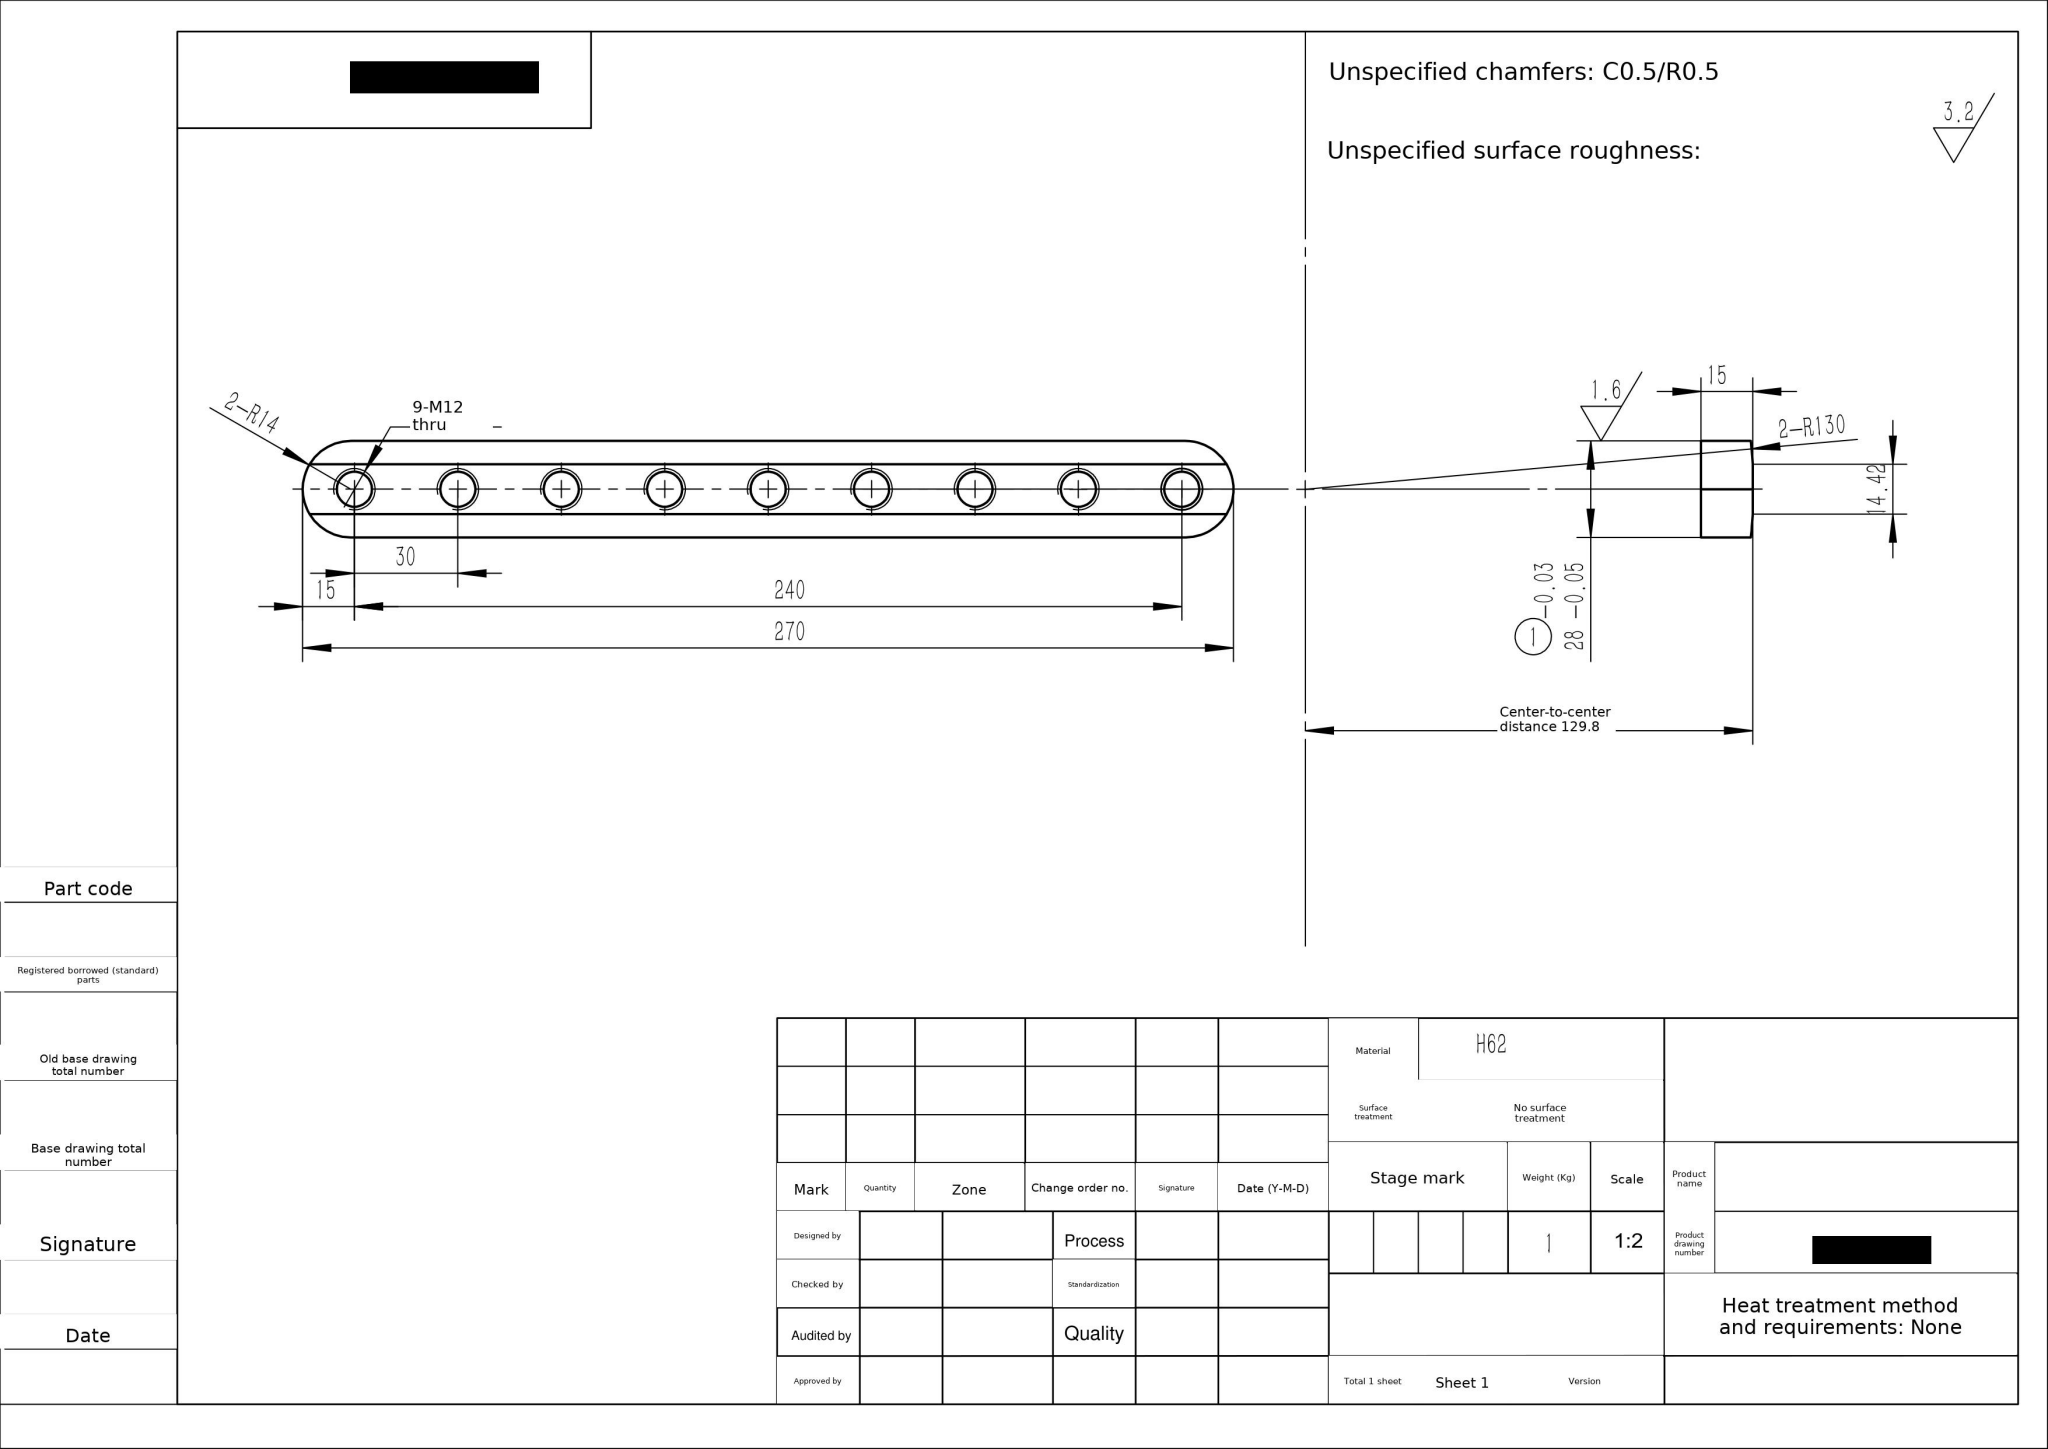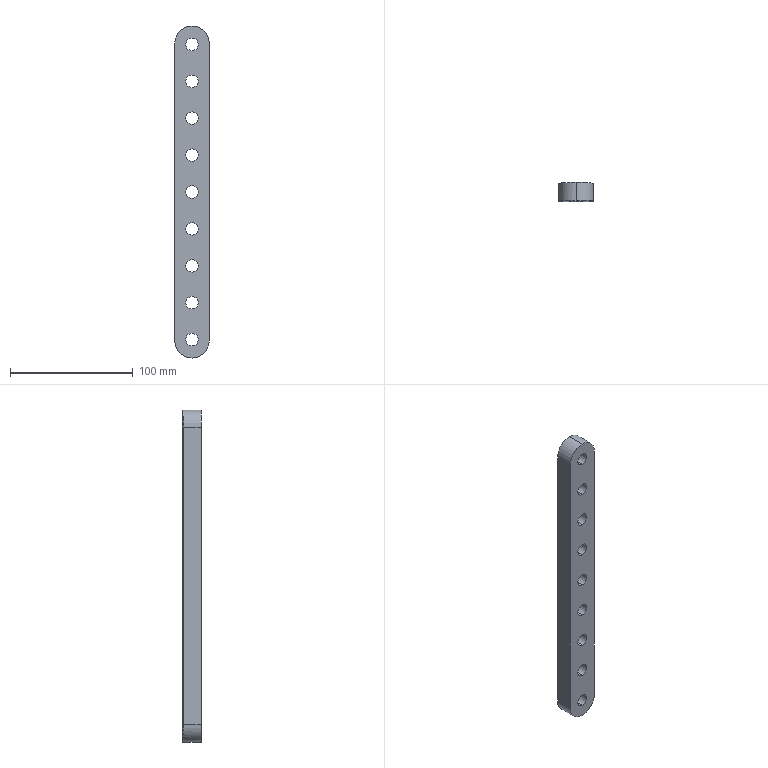Part | SolidWorks | mm | material H62 | 1 solid | 28 faces | box 28 x 15 x 270 mm | volume 98984 mm3 | cylinder 24 | plane 4 | commonest cylinder face diameters 10.2 x18 28 x4 260 x2
STEP:
#1=CARTESIAN_POINT('',(0.,-7.5,-125.1));
#2=VERTEX_POINT('',#1);
#3=CARTESIAN_POINT('',(0.,-7.5,-114.9));
#4=VERTEX_POINT('',#3);
#5=CARTESIAN_POINT('',(0.,-7.5,-120.));
#6=DIRECTION('',(0.,1.,0.));
#7=DIRECTION('',(0.,0.,1.));
#8=AXIS2_PLACEMENT_3D('',#5,#6,#7);
#9=CIRCLE('',#8,5.1);
#10=EDGE_CURVE('',#2,#4,#9,.T.);
#11=ORIENTED_EDGE('',*,*,#10,.F.);
#12=CARTESIAN_POINT('',(0.,7.5,-125.1));
#13=VERTEX_POINT('',#12);
#14=CARTESIAN_POINT('',(0.,7.5,-125.1));
#15=DIRECTION('',(0.,1.,0.));
#16=VECTOR('',#15,1000.);
#17=LINE('',#14,#16);
#18=EDGE_CURVE('',#2,#13,#17,.T.);
#19=ORIENTED_EDGE('',*,*,#18,.T.);
#20=CARTESIAN_POINT('',(0.,7.5,-114.9));
#21=VERTEX_POINT('',#20);
#22=CARTESIAN_POINT('',(0.,7.5,-120.));
#23=DIRECTION('',(0.,1.,0.));
#24=DIRECTION('',(0.,0.,1.));
#25=AXIS2_PLACEMENT_3D('',#22,#23,#24);
#26=CIRCLE('',#25,5.1);
#27=EDGE_CURVE('',#13,#21,#26,.T.);
#28=ORIENTED_EDGE('',*,*,#27,.T.);
#29=CARTESIAN_POINT('',(0.,7.5,-114.9));
#30=DIRECTION('',(0.,1.,0.));
#31=VECTOR('',#30,1000.);
#32=LINE('',#29,#31);
#33=EDGE_CURVE('',#4,#21,#32,.T.);
#34=ORIENTED_EDGE('',*,*,#33,.F.);
#35=EDGE_LOOP('',(#11,#19,#28,#34));
#36=FACE_OUTER_BOUND('',#35,.T.);
#37=CARTESIAN_POINT('',(0.,7.5,-120.));
#38=DIRECTION('',(0.,1.,0.));
#39=DIRECTION('',(0.,0.,1.));
#40=AXIS2_PLACEMENT_3D('',#37,#38,#39);
#41=CYLINDRICAL_SURFACE('',#40,5.1);
#42=ADVANCED_FACE('',(#36),#41,.F.);
#43=CARTESIAN_POINT('',(0.,-7.5,-95.1));
#44=VERTEX_POINT('',#43);
#45=CARTESIAN_POINT('',(0.,-7.5,-84.9));
#46=VERTEX_POINT('',#45);
#47=CARTESIAN_POINT('',(0.,-7.5,-90.));
#48=DIRECTION('',(0.,1.,0.));
#49=DIRECTION('',(0.,0.,1.));
#50=AXIS2_PLACEMENT_3D('',#47,#48,#49);
#51=CIRCLE('',#50,5.1);
#52=EDGE_CURVE('',#44,#46,#51,.T.);
#53=ORIENTED_EDGE('',*,*,#52,.F.);
#54=CARTESIAN_POINT('',(0.,7.5,-95.1));
#55=VERTEX_POINT('',#54);
#56=CARTESIAN_POINT('',(0.,7.5,-95.1));
#57=DIRECTION('',(0.,1.,0.));
#58=VECTOR('',#57,1000.);
#59=LINE('',#56,#58);
#60=EDGE_CURVE('',#44,#55,#59,.T.);
#61=ORIENTED_EDGE('',*,*,#60,.T.);
#62=CARTESIAN_POINT('',(0.,7.5,-84.9));
#63=VERTEX_POINT('',#62);
#64=CARTESIAN_POINT('',(0.,7.5,-90.));
#65=DIRECTION('',(0.,1.,0.));
#66=DIRECTION('',(0.,0.,1.));
#67=AXIS2_PLACEMENT_3D('',#64,#65,#66);
#68=CIRCLE('',#67,5.1);
#69=EDGE_CURVE('',#55,#63,#68,.T.);
#70=ORIENTED_EDGE('',*,*,#69,.T.);
#71=CARTESIAN_POINT('',(0.,7.5,-84.9));
#72=DIRECTION('',(0.,1.,0.));
#73=VECTOR('',#72,1000.);
#74=LINE('',#71,#73);
#75=EDGE_CURVE('',#46,#63,#74,.T.);
#76=ORIENTED_EDGE('',*,*,#75,.F.);
#77=EDGE_LOOP('',(#53,#61,#70,#76));
#78=FACE_OUTER_BOUND('',#77,.T.);
#79=CARTESIAN_POINT('',(0.,7.5,-90.));
#80=DIRECTION('',(0.,1.,0.));
#81=DIRECTION('',(0.,0.,1.));
#82=AXIS2_PLACEMENT_3D('',#79,#80,#81);
#83=CYLINDRICAL_SURFACE('',#82,5.1);
#84=ADVANCED_FACE('',(#78),#83,.F.);
#85=CARTESIAN_POINT('',(0.,-7.5,-65.1));
#86=VERTEX_POINT('',#85);
#87=CARTESIAN_POINT('',(0.,-7.5,-54.9));
#88=VERTEX_POINT('',#87);
#89=CARTESIAN_POINT('',(0.,-7.5,-60.));
#90=DIRECTION('',(0.,1.,0.));
#91=DIRECTION('',(0.,0.,1.));
#92=AXIS2_PLACEMENT_3D('',#89,#90,#91);
#93=CIRCLE('',#92,5.1);
#94=EDGE_CURVE('',#86,#88,#93,.T.);
#95=ORIENTED_EDGE('',*,*,#94,.F.);
#96=CARTESIAN_POINT('',(0.,7.5,-65.1));
#97=VERTEX_POINT('',#96);
#98=CARTESIAN_POINT('',(0.,7.5,-65.1));
#99=DIRECTION('',(0.,1.,0.));
#100=VECTOR('',#99,1000.);
#101=LINE('',#98,#100);
#102=EDGE_CURVE('',#86,#97,#101,.T.);
#103=ORIENTED_EDGE('',*,*,#102,.T.);
#104=CARTESIAN_POINT('',(0.,7.5,-54.9));
#105=VERTEX_POINT('',#104);
#106=CARTESIAN_POINT('',(0.,7.5,-60.));
#107=DIRECTION('',(0.,1.,0.));
#108=DIRECTION('',(0.,0.,1.));
#109=AXIS2_PLACEMENT_3D('',#106,#107,#108);
#110=CIRCLE('',#109,5.1);
#111=EDGE_CURVE('',#97,#105,#110,.T.);
#112=ORIENTED_EDGE('',*,*,#111,.T.);
#113=CARTESIAN_POINT('',(0.,7.5,-54.9));
#114=DIRECTION('',(0.,1.,0.));
#115=VECTOR('',#114,1000.);
#116=LINE('',#113,#115);
#117=EDGE_CURVE('',#88,#105,#116,.T.);
#118=ORIENTED_EDGE('',*,*,#117,.F.);
#119=EDGE_LOOP('',(#95,#103,#112,#118));
#120=FACE_OUTER_BOUND('',#119,.T.);
#121=CARTESIAN_POINT('',(0.,7.5,-60.));
#122=DIRECTION('',(0.,1.,0.));
#123=DIRECTION('',(0.,0.,1.));
#124=AXIS2_PLACEMENT_3D('',#121,#122,#123);
#125=CYLINDRICAL_SURFACE('',#124,5.1);
#126=ADVANCED_FACE('',(#120),#125,.F.);
#127=CARTESIAN_POINT('',(0.,-7.5,-35.1));
#128=VERTEX_POINT('',#127);
#129=CARTESIAN_POINT('',(0.,-7.5,-24.9));
#130=VERTEX_POINT('',#129);
#131=CARTESIAN_POINT('',(0.,-7.5,-30.));
#132=DIRECTION('',(0.,1.,0.));
#133=DIRECTION('',(0.,0.,1.));
#134=AXIS2_PLACEMENT_3D('',#131,#132,#133);
#135=CIRCLE('',#134,5.1);
#136=EDGE_CURVE('',#128,#130,#135,.T.);
#137=ORIENTED_EDGE('',*,*,#136,.F.);
#138=CARTESIAN_POINT('',(0.,7.5,-35.1));
#139=VERTEX_POINT('',#138);
#140=CARTESIAN_POINT('',(0.,7.5,-35.1));
#141=DIRECTION('',(0.,1.,0.));
#142=VECTOR('',#141,1000.);
#143=LINE('',#140,#142);
#144=EDGE_CURVE('',#128,#139,#143,.T.);
#145=ORIENTED_EDGE('',*,*,#144,.T.);
#146=CARTESIAN_POINT('',(0.,7.5,-24.9));
#147=VERTEX_POINT('',#146);
#148=CARTESIAN_POINT('',(0.,7.5,-30.));
#149=DIRECTION('',(0.,1.,0.));
#150=DIRECTION('',(0.,0.,1.));
#151=AXIS2_PLACEMENT_3D('',#148,#149,#150);
#152=CIRCLE('',#151,5.1);
#153=EDGE_CURVE('',#139,#147,#152,.T.);
#154=ORIENTED_EDGE('',*,*,#153,.T.);
#155=CARTESIAN_POINT('',(0.,7.5,-24.9));
#156=DIRECTION('',(0.,1.,0.));
#157=VECTOR('',#156,1000.);
#158=LINE('',#155,#157);
#159=EDGE_CURVE('',#130,#147,#158,.T.);
#160=ORIENTED_EDGE('',*,*,#159,.F.);
#161=EDGE_LOOP('',(#137,#145,#154,#160));
#162=FACE_OUTER_BOUND('',#161,.T.);
#163=CARTESIAN_POINT('',(0.,7.5,-30.));
#164=DIRECTION('',(0.,1.,0.));
#165=DIRECTION('',(0.,0.,1.));
#166=AXIS2_PLACEMENT_3D('',#163,#164,#165);
#167=CYLINDRICAL_SURFACE('',#166,5.1);
#168=ADVANCED_FACE('',(#162),#167,.F.);
#169=CARTESIAN_POINT('',(0.,-7.5,-5.1));
#170=VERTEX_POINT('',#169);
#171=CARTESIAN_POINT('',(0.,-7.5,5.1));
#172=VERTEX_POINT('',#171);
#173=CARTESIAN_POINT('',(0.,-7.5,0.));
#174=DIRECTION('',(0.,1.,0.));
#175=DIRECTION('',(0.,0.,1.));
#176=AXIS2_PLACEMENT_3D('',#173,#174,#175);
#177=CIRCLE('',#176,5.1);
#178=EDGE_CURVE('',#170,#172,#177,.T.);
#179=ORIENTED_EDGE('',*,*,#178,.F.);
#180=CARTESIAN_POINT('',(0.,7.5,-5.1));
#181=VERTEX_POINT('',#180);
#182=CARTESIAN_POINT('',(0.,7.5,-5.1));
#183=DIRECTION('',(0.,1.,0.));
#184=VECTOR('',#183,1000.);
#185=LINE('',#182,#184);
#186=EDGE_CURVE('',#170,#181,#185,.T.);
#187=ORIENTED_EDGE('',*,*,#186,.T.);
#188=CARTESIAN_POINT('',(0.,7.5,5.1));
#189=VERTEX_POINT('',#188);
#190=CARTESIAN_POINT('',(0.,7.5,0.));
#191=DIRECTION('',(0.,1.,0.));
#192=DIRECTION('',(0.,0.,1.));
#193=AXIS2_PLACEMENT_3D('',#190,#191,#192);
#194=CIRCLE('',#193,5.1);
#195=EDGE_CURVE('',#181,#189,#194,.T.);
#196=ORIENTED_EDGE('',*,*,#195,.T.);
#197=CARTESIAN_POINT('',(0.,7.5,5.1));
#198=DIRECTION('',(0.,1.,0.));
#199=VECTOR('',#198,1000.);
#200=LINE('',#197,#199);
#201=EDGE_CURVE('',#172,#189,#200,.T.);
#202=ORIENTED_EDGE('',*,*,#201,.F.);
#203=EDGE_LOOP('',(#179,#187,#196,#202));
#204=FACE_OUTER_BOUND('',#203,.T.);
#205=CARTESIAN_POINT('',(0.,7.5,0.));
#206=DIRECTION('',(0.,1.,0.));
#207=DIRECTION('',(0.,0.,1.));
#208=AXIS2_PLACEMENT_3D('',#205,#206,#207);
#209=CYLINDRICAL_SURFACE('',#208,5.1);
#210=ADVANCED_FACE('',(#204),#209,.F.);
#211=CARTESIAN_POINT('',(0.,-7.5,24.9));
#212=VERTEX_POINT('',#211);
#213=CARTESIAN_POINT('',(0.,-7.5,35.1));
#214=VERTEX_POINT('',#213);
#215=CARTESIAN_POINT('',(0.,-7.5,30.));
#216=DIRECTION('',(0.,1.,0.));
#217=DIRECTION('',(0.,0.,1.));
#218=AXIS2_PLACEMENT_3D('',#215,#216,#217);
#219=CIRCLE('',#218,5.1);
#220=EDGE_CURVE('',#212,#214,#219,.T.);
#221=ORIENTED_EDGE('',*,*,#220,.F.);
#222=CARTESIAN_POINT('',(0.,7.5,24.9));
#223=VERTEX_POINT('',#222);
#224=CARTESIAN_POINT('',(0.,7.5,24.9));
#225=DIRECTION('',(0.,1.,0.));
#226=VECTOR('',#225,1000.);
#227=LINE('',#224,#226);
#228=EDGE_CURVE('',#212,#223,#227,.T.);
#229=ORIENTED_EDGE('',*,*,#228,.T.);
#230=CARTESIAN_POINT('',(0.,7.5,35.1));
#231=VERTEX_POINT('',#230);
#232=CARTESIAN_POINT('',(0.,7.5,30.));
#233=DIRECTION('',(0.,1.,0.));
#234=DIRECTION('',(0.,0.,1.));
#235=AXIS2_PLACEMENT_3D('',#232,#233,#234);
#236=CIRCLE('',#235,5.1);
#237=EDGE_CURVE('',#223,#231,#236,.T.);
#238=ORIENTED_EDGE('',*,*,#237,.T.);
#239=CARTESIAN_POINT('',(0.,7.5,35.1));
#240=DIRECTION('',(0.,1.,0.));
#241=VECTOR('',#240,1000.);
#242=LINE('',#239,#241);
#243=EDGE_CURVE('',#214,#231,#242,.T.);
#244=ORIENTED_EDGE('',*,*,#243,.F.);
#245=EDGE_LOOP('',(#221,#229,#238,#244));
#246=FACE_OUTER_BOUND('',#245,.T.);
#247=CARTESIAN_POINT('',(0.,7.5,30.));
#248=DIRECTION('',(0.,1.,0.));
#249=DIRECTION('',(0.,0.,1.));
#250=AXIS2_PLACEMENT_3D('',#247,#248,#249);
#251=CYLINDRICAL_SURFACE('',#250,5.1);
#252=ADVANCED_FACE('',(#246),#251,.F.);
#253=CARTESIAN_POINT('',(0.,-7.5,54.9));
#254=VERTEX_POINT('',#253);
#255=CARTESIAN_POINT('',(0.,-7.5,65.1));
#256=VERTEX_POINT('',#255);
#257=CARTESIAN_POINT('',(0.,-7.5,60.));
#258=DIRECTION('',(0.,1.,0.));
#259=DIRECTION('',(0.,0.,1.));
#260=AXIS2_PLACEMENT_3D('',#257,#258,#259);
#261=CIRCLE('',#260,5.1);
#262=EDGE_CURVE('',#254,#256,#261,.T.);
#263=ORIENTED_EDGE('',*,*,#262,.F.);
#264=CARTESIAN_POINT('',(0.,7.5,54.9));
#265=VERTEX_POINT('',#264);
#266=CARTESIAN_POINT('',(0.,7.5,54.9));
#267=DIRECTION('',(0.,1.,0.));
#268=VECTOR('',#267,1000.);
#269=LINE('',#266,#268);
#270=EDGE_CURVE('',#254,#265,#269,.T.);
#271=ORIENTED_EDGE('',*,*,#270,.T.);
#272=CARTESIAN_POINT('',(0.,7.5,65.1));
#273=VERTEX_POINT('',#272);
#274=CARTESIAN_POINT('',(0.,7.5,60.));
#275=DIRECTION('',(0.,1.,0.));
#276=DIRECTION('',(0.,0.,1.));
#277=AXIS2_PLACEMENT_3D('',#274,#275,#276);
#278=CIRCLE('',#277,5.1);
#279=EDGE_CURVE('',#265,#273,#278,.T.);
#280=ORIENTED_EDGE('',*,*,#279,.T.);
#281=CARTESIAN_POINT('',(0.,7.5,65.1));
#282=DIRECTION('',(0.,1.,0.));
#283=VECTOR('',#282,1000.);
#284=LINE('',#281,#283);
#285=EDGE_CURVE('',#256,#273,#284,.T.);
#286=ORIENTED_EDGE('',*,*,#285,.F.);
#287=EDGE_LOOP('',(#263,#271,#280,#286));
#288=FACE_OUTER_BOUND('',#287,.T.);
#289=CARTESIAN_POINT('',(0.,7.5,60.));
#290=DIRECTION('',(0.,1.,0.));
#291=DIRECTION('',(0.,0.,1.));
#292=AXIS2_PLACEMENT_3D('',#289,#290,#291);
#293=CYLINDRICAL_SURFACE('',#292,5.1);
#294=ADVANCED_FACE('',(#288),#293,.F.);
#295=CARTESIAN_POINT('',(0.,-7.5,84.9));
#296=VERTEX_POINT('',#295);
#297=CARTESIAN_POINT('',(0.,-7.5,95.1));
#298=VERTEX_POINT('',#297);
#299=CARTESIAN_POINT('',(0.,-7.5,90.));
#300=DIRECTION('',(0.,1.,0.));
#301=DIRECTION('',(0.,0.,1.));
#302=AXIS2_PLACEMENT_3D('',#299,#300,#301);
#303=CIRCLE('',#302,5.1);
#304=EDGE_CURVE('',#296,#298,#303,.T.);
#305=ORIENTED_EDGE('',*,*,#304,.F.);
#306=CARTESIAN_POINT('',(0.,7.5,84.9));
#307=VERTEX_POINT('',#306);
#308=CARTESIAN_POINT('',(0.,7.5,84.9));
#309=DIRECTION('',(0.,1.,0.));
#310=VECTOR('',#309,1000.);
#311=LINE('',#308,#310);
#312=EDGE_CURVE('',#296,#307,#311,.T.);
#313=ORIENTED_EDGE('',*,*,#312,.T.);
#314=CARTESIAN_POINT('',(0.,7.5,95.1));
#315=VERTEX_POINT('',#314);
#316=CARTESIAN_POINT('',(0.,7.5,90.));
#317=DIRECTION('',(0.,1.,0.));
#318=DIRECTION('',(0.,0.,1.));
#319=AXIS2_PLACEMENT_3D('',#316,#317,#318);
#320=CIRCLE('',#319,5.1);
#321=EDGE_CURVE('',#307,#315,#320,.T.);
#322=ORIENTED_EDGE('',*,*,#321,.T.);
#323=CARTESIAN_POINT('',(0.,7.5,95.1));
#324=DIRECTION('',(0.,1.,0.));
#325=VECTOR('',#324,1000.);
#326=LINE('',#323,#325);
#327=EDGE_CURVE('',#298,#315,#326,.T.);
#328=ORIENTED_EDGE('',*,*,#327,.F.);
#329=EDGE_LOOP('',(#305,#313,#322,#328));
#330=FACE_OUTER_BOUND('',#329,.T.);
#331=CARTESIAN_POINT('',(0.,7.5,90.));
#332=DIRECTION('',(0.,1.,0.));
#333=DIRECTION('',(0.,0.,1.));
#334=AXIS2_PLACEMENT_3D('',#331,#332,#333);
#335=CYLINDRICAL_SURFACE('',#334,5.1);
#336=ADVANCED_FACE('',(#330),#335,.F.);
#337=CARTESIAN_POINT('',(0.,-7.5,114.9));
#338=VERTEX_POINT('',#337);
#339=CARTESIAN_POINT('',(0.,-7.5,125.1));
#340=VERTEX_POINT('',#339);
#341=CARTESIAN_POINT('',(0.,-7.5,120.));
#342=DIRECTION('',(0.,1.,0.));
#343=DIRECTION('',(0.,0.,1.));
#344=AXIS2_PLACEMENT_3D('',#341,#342,#343);
#345=CIRCLE('',#344,5.1);
#346=EDGE_CURVE('',#338,#340,#345,.T.);
#347=ORIENTED_EDGE('',*,*,#346,.F.);
#348=CARTESIAN_POINT('',(0.,7.5,114.9));
#349=VERTEX_POINT('',#348);
#350=CARTESIAN_POINT('',(0.,7.5,114.9));
#351=DIRECTION('',(0.,1.,0.));
#352=VECTOR('',#351,1000.);
#353=LINE('',#350,#352);
#354=EDGE_CURVE('',#338,#349,#353,.T.);
#355=ORIENTED_EDGE('',*,*,#354,.T.);
#356=CARTESIAN_POINT('',(0.,7.5,125.1));
#357=VERTEX_POINT('',#356);
#358=CARTESIAN_POINT('',(0.,7.5,120.));
#359=DIRECTION('',(0.,1.,0.));
#360=DIRECTION('',(0.,0.,1.));
#361=AXIS2_PLACEMENT_3D('',#358,#359,#360);
#362=CIRCLE('',#361,5.1);
#363=EDGE_CURVE('',#349,#357,#362,.T.);
#364=ORIENTED_EDGE('',*,*,#363,.T.);
#365=CARTESIAN_POINT('',(0.,7.5,125.1));
#366=DIRECTION('',(0.,1.,0.));
#367=VECTOR('',#366,1000.);
#368=LINE('',#365,#367);
#369=EDGE_CURVE('',#340,#357,#368,.T.);
#370=ORIENTED_EDGE('',*,*,#369,.F.);
#371=EDGE_LOOP('',(#347,#355,#364,#370));
#372=FACE_OUTER_BOUND('',#371,.T.);
#373=CARTESIAN_POINT('',(0.,7.5,120.));
#374=DIRECTION('',(0.,1.,0.));
#375=DIRECTION('',(0.,0.,1.));
#376=AXIS2_PLACEMENT_3D('',#373,#374,#375);
#377=CYLINDRICAL_SURFACE('',#376,5.1);
#378=ADVANCED_FACE('',(#372),#377,.F.);
#379=CARTESIAN_POINT('',(0.,7.5,-120.));
#380=DIRECTION('',(0.,1.,0.));
#381=DIRECTION('',(0.,0.,1.));
#382=AXIS2_PLACEMENT_3D('',#379,#380,#381);
#383=CIRCLE('',#382,5.1);
#384=EDGE_CURVE('',#21,#13,#383,.T.);
#385=ORIENTED_EDGE('',*,*,#384,.F.);
#386=ORIENTED_EDGE('',*,*,#27,.F.);
#387=EDGE_LOOP('',(#385,#386));
#388=FACE_BOUND('',#387,.T.);
#389=CARTESIAN_POINT('',(0.,7.5,-90.));
#390=DIRECTION('',(0.,1.,0.));
#391=DIRECTION('',(0.,0.,1.));
#392=AXIS2_PLACEMENT_3D('',#389,#390,#391);
#393=CIRCLE('',#392,5.1);
#394=EDGE_CURVE('',#63,#55,#393,.T.);
#395=ORIENTED_EDGE('',*,*,#394,.F.);
#396=ORIENTED_EDGE('',*,*,#69,.F.);
#397=EDGE_LOOP('',(#395,#396));
#398=FACE_BOUND('',#397,.T.);
#399=CARTESIAN_POINT('',(0.,7.5,-60.));
#400=DIRECTION('',(0.,1.,0.));
#401=DIRECTION('',(0.,0.,1.));
#402=AXIS2_PLACEMENT_3D('',#399,#400,#401);
#403=CIRCLE('',#402,5.1);
#404=EDGE_CURVE('',#105,#97,#403,.T.);
#405=ORIENTED_EDGE('',*,*,#404,.F.);
#406=ORIENTED_EDGE('',*,*,#111,.F.);
#407=EDGE_LOOP('',(#405,#406));
#408=FACE_BOUND('',#407,.T.);
#409=CARTESIAN_POINT('',(0.,7.5,-30.));
#410=DIRECTION('',(0.,1.,0.));
#411=DIRECTION('',(0.,0.,1.));
#412=AXIS2_PLACEMENT_3D('',#409,#410,#411);
#413=CIRCLE('',#412,5.1);
#414=EDGE_CURVE('',#147,#139,#413,.T.);
#415=ORIENTED_EDGE('',*,*,#414,.F.);
#416=ORIENTED_EDGE('',*,*,#153,.F.);
#417=EDGE_LOOP('',(#415,#416));
#418=FACE_BOUND('',#417,.T.);
#419=CARTESIAN_POINT('',(0.,7.5,0.));
#420=DIRECTION('',(0.,1.,0.));
#421=DIRECTION('',(0.,0.,1.));
#422=AXIS2_PLACEMENT_3D('',#419,#420,#421);
#423=CIRCLE('',#422,5.1);
#424=EDGE_CURVE('',#189,#181,#423,.T.);
#425=ORIENTED_EDGE('',*,*,#424,.F.);
#426=ORIENTED_EDGE('',*,*,#195,.F.);
#427=EDGE_LOOP('',(#425,#426));
#428=FACE_BOUND('',#427,.T.);
#429=CARTESIAN_POINT('',(0.,7.5,60.));
#430=DIRECTION('',(0.,1.,0.));
#431=DIRECTION('',(0.,0.,1.));
#432=AXIS2_PLACEMENT_3D('',#429,#430,#431);
#433=CIRCLE('',#432,5.1);
#434=EDGE_CURVE('',#273,#265,#433,.T.);
#435=ORIENTED_EDGE('',*,*,#434,.F.);
#436=ORIENTED_EDGE('',*,*,#279,.F.);
#437=EDGE_LOOP('',(#435,#436));
#438=FACE_BOUND('',#437,.T.);
#439=CARTESIAN_POINT('',(0.,7.5,90.));
#440=DIRECTION('',(0.,1.,0.));
#441=DIRECTION('',(0.,0.,1.));
#442=AXIS2_PLACEMENT_3D('',#439,#440,#441);
#443=CIRCLE('',#442,5.1);
#444=EDGE_CURVE('',#315,#307,#443,.T.);
#445=ORIENTED_EDGE('',*,*,#444,.F.);
#446=ORIENTED_EDGE('',*,*,#321,.F.);
#447=EDGE_LOOP('',(#445,#446));
#448=FACE_BOUND('',#447,.T.);
#449=CARTESIAN_POINT('',(0.,7.5,120.));
#450=DIRECTION('',(0.,1.,0.));
#451=DIRECTION('',(0.,0.,1.));
#452=AXIS2_PLACEMENT_3D('',#449,#450,#451);
#453=CIRCLE('',#452,5.1);
#454=EDGE_CURVE('',#357,#349,#453,.T.);
#455=ORIENTED_EDGE('',*,*,#454,.F.);
#456=ORIENTED_EDGE('',*,*,#363,.F.);
#457=EDGE_LOOP('',(#455,#456));
#458=FACE_BOUND('',#457,.T.);
#459=CARTESIAN_POINT('',(7.208,7.5,-133.002));
#460=VERTEX_POINT('',#459);
#461=CARTESIAN_POINT('',(-0.,7.5,-135.));
#462=VERTEX_POINT('',#461);
#463=CARTESIAN_POINT('',(-0.,7.5,-121.));
#464=DIRECTION('',(0.,1.,0.));
#465=DIRECTION('',(0.,0.,-1.));
#466=AXIS2_PLACEMENT_3D('',#463,#464,#465);
#467=CIRCLE('',#466,14.);
#468=EDGE_CURVE('',#460,#462,#467,.T.);
#469=ORIENTED_EDGE('',*,*,#468,.T.);
#470=CARTESIAN_POINT('',(-7.208,7.5,-133.002));
#471=VERTEX_POINT('',#470);
#472=CARTESIAN_POINT('',(-0.,7.5,-121.));
#473=DIRECTION('',(0.,1.,0.));
#474=DIRECTION('',(0.,0.,-1.));
#475=AXIS2_PLACEMENT_3D('',#472,#473,#474);
#476=CIRCLE('',#475,14.);
#477=EDGE_CURVE('',#462,#471,#476,.T.);
#478=ORIENTED_EDGE('',*,*,#477,.T.);
#479=CARTESIAN_POINT('',(-7.208,7.5,133.002));
#480=VERTEX_POINT('',#479);
#481=CARTESIAN_POINT('',(-7.208,7.5,-135.));
#482=DIRECTION('',(0.,0.,-1.));
#483=VECTOR('',#482,1000.);
#484=LINE('',#481,#483);
#485=EDGE_CURVE('',#480,#471,#484,.T.);
#486=ORIENTED_EDGE('',*,*,#485,.F.);
#487=CARTESIAN_POINT('',(-0.,7.5,135.));
#488=VERTEX_POINT('',#487);
#489=CARTESIAN_POINT('',(-0.,7.5,121.));
#490=DIRECTION('',(0.,1.,0.));
#491=DIRECTION('',(0.,0.,-1.));
#492=AXIS2_PLACEMENT_3D('',#489,#490,#491);
#493=CIRCLE('',#492,14.);
#494=EDGE_CURVE('',#480,#488,#493,.T.);
#495=ORIENTED_EDGE('',*,*,#494,.T.);
#496=CARTESIAN_POINT('',(7.208,7.5,133.002));
#497=VERTEX_POINT('',#496);
#498=CARTESIAN_POINT('',(-0.,7.5,121.));
#499=DIRECTION('',(0.,1.,0.));
#500=DIRECTION('',(-0.,0.,-1.));
#501=AXIS2_PLACEMENT_3D('',#498,#499,#500);
#502=CIRCLE('',#501,14.);
#503=EDGE_CURVE('',#488,#497,#502,.T.);
#504=ORIENTED_EDGE('',*,*,#503,.T.);
#505=CARTESIAN_POINT('',(7.208,7.5,-135.));
#506=DIRECTION('',(0.,0.,1.));
#507=VECTOR('',#506,1000.);
#508=LINE('',#505,#507);
#509=EDGE_CURVE('',#460,#497,#508,.T.);
#510=ORIENTED_EDGE('',*,*,#509,.F.);
#511=EDGE_LOOP('',(#469,#478,#486,#495,#504,#510));
#512=FACE_OUTER_BOUND('',#511,.T.);
#513=CARTESIAN_POINT('',(0.,7.5,30.));
#514=DIRECTION('',(0.,1.,0.));
#515=DIRECTION('',(0.,0.,1.));
#516=AXIS2_PLACEMENT_3D('',#513,#514,#515);
#517=CIRCLE('',#516,5.1);
#518=EDGE_CURVE('',#231,#223,#517,.T.);
#519=ORIENTED_EDGE('',*,*,#518,.F.);
#520=ORIENTED_EDGE('',*,*,#237,.F.);
#521=EDGE_LOOP('',(#519,#520));
#522=FACE_BOUND('',#521,.T.);
#523=CARTESIAN_POINT('',(-14.,7.5,135.));
#524=DIRECTION('',(0.,-1.,0.));
#525=DIRECTION('',(0.,0.,-1.));
#526=AXIS2_PLACEMENT_3D('',#523,#524,#525);
#527=PLANE('',#526);
#528=ADVANCED_FACE('',(#388,#398,#408,#418,#428,#438,#448,#458,#512,#522),#527,.F.);
#529=CARTESIAN_POINT('',(14.,-7.5,121.));
#530=VERTEX_POINT('',#529);
#531=CARTESIAN_POINT('',(14.,-7.5,-121.));
#532=VERTEX_POINT('',#531);
#533=CARTESIAN_POINT('',(14.,-7.5,135.));
#534=DIRECTION('',(0.,0.,-1.));
#535=VECTOR('',#534,1000.);
#536=LINE('',#533,#535);
#537=EDGE_CURVE('',#530,#532,#536,.T.);
#538=ORIENTED_EDGE('',*,*,#537,.T.);
#539=CARTESIAN_POINT('',(14.,6.944,-121.));
#540=VERTEX_POINT('',#539);
#541=CARTESIAN_POINT('',(14.,7.5,-121.));
#542=DIRECTION('',(-0.,1.,0.));
#543=VECTOR('',#542,1000.);
#544=LINE('',#541,#543);
#545=EDGE_CURVE('',#532,#540,#544,.T.);
#546=ORIENTED_EDGE('',*,*,#545,.T.);
#547=CARTESIAN_POINT('',(14.,6.944,121.));
#548=VERTEX_POINT('',#547);
#549=CARTESIAN_POINT('',(14.,6.944,-135.));
#550=DIRECTION('',(0.,0.,-1.));
#551=VECTOR('',#550,1000.);
#552=LINE('',#549,#551);
#553=EDGE_CURVE('',#548,#540,#552,.T.);
#554=ORIENTED_EDGE('',*,*,#553,.F.);
#555=CARTESIAN_POINT('',(14.,-7.5,121.));
#556=DIRECTION('',(0.,-1.,0.));
#557=VECTOR('',#556,1000.);
#558=LINE('',#555,#557);
#559=EDGE_CURVE('',#548,#530,#558,.T.);
#560=ORIENTED_EDGE('',*,*,#559,.T.);
#561=EDGE_LOOP('',(#538,#546,#554,#560));
#562=FACE_OUTER_BOUND('',#561,.T.);
#563=CARTESIAN_POINT('',(14.,7.5,135.));
#564=DIRECTION('',(-1.,-0.,0.));
#565=DIRECTION('',(0.,-1.,0.));
#566=AXIS2_PLACEMENT_3D('',#563,#564,#565);
#567=PLANE('',#566);
#568=ADVANCED_FACE('',(#562),#567,.F.);
#569=CARTESIAN_POINT('',(-14.,6.944,-121.));
#570=VERTEX_POINT('',#569);
#571=CARTESIAN_POINT('',(-14.,6.944,121.));
#572=VERTEX_POINT('',#571);
#573=CARTESIAN_POINT('',(-14.,6.944,-135.));
#574=DIRECTION('',(0.,0.,1.));
#575=VECTOR('',#574,1000.);
#576=LINE('',#573,#575);
#577=EDGE_CURVE('',#570,#572,#576,.T.);
#578=ORIENTED_EDGE('',*,*,#577,.F.);
#579=CARTESIAN_POINT('',(-14.,-7.5,-121.));
#580=VERTEX_POINT('',#579);
#581=CARTESIAN_POINT('',(-14.,7.5,-121.));
#582=DIRECTION('',(0.,-1.,0.));
#583=VECTOR('',#582,1000.);
#584=LINE('',#581,#583);
#585=EDGE_CURVE('',#570,#580,#584,.T.);
#586=ORIENTED_EDGE('',*,*,#585,.T.);
#587=CARTESIAN_POINT('',(-14.,-7.5,121.));
#588=VERTEX_POINT('',#587);
#589=CARTESIAN_POINT('',(-14.,-7.5,135.));
#590=DIRECTION('',(0.,0.,-1.));
#591=VECTOR('',#590,1000.);
#592=LINE('',#589,#591);
#593=EDGE_CURVE('',#588,#580,#592,.T.);
#594=ORIENTED_EDGE('',*,*,#593,.F.);
#595=CARTESIAN_POINT('',(-14.,6.944,121.));
#596=DIRECTION('',(-0.,1.,0.));
#597=VECTOR('',#596,1000.);
#598=LINE('',#595,#597);
#599=EDGE_CURVE('',#588,#572,#598,.T.);
#600=ORIENTED_EDGE('',*,*,#599,.T.);
#601=EDGE_LOOP('',(#578,#586,#594,#600));
#602=FACE_OUTER_BOUND('',#601,.T.);
#603=CARTESIAN_POINT('',(-14.,7.5,135.));
#604=DIRECTION('',(1.,0.,0.));
#605=DIRECTION('',(-0.,1.,0.));
#606=AXIS2_PLACEMENT_3D('',#603,#604,#605);
#607=PLANE('',#606);
#608=ADVANCED_FACE('',(#602),#607,.F.);
#609=CARTESIAN_POINT('',(0.,-7.5,-120.));
#610=DIRECTION('',(0.,1.,0.));
#611=DIRECTION('',(0.,0.,1.));
#612=AXIS2_PLACEMENT_3D('',#609,#610,#611);
#613=CIRCLE('',#612,5.1);
#614=EDGE_CURVE('',#4,#2,#613,.T.);
#615=ORIENTED_EDGE('',*,*,#614,.T.);
#616=ORIENTED_EDGE('',*,*,#10,.T.);
#617=EDGE_LOOP('',(#615,#616));
#618=FACE_BOUND('',#617,.T.);
#619=CARTESIAN_POINT('',(0.,-7.5,-90.));
#620=DIRECTION('',(0.,1.,0.));
#621=DIRECTION('',(0.,0.,1.));
#622=AXIS2_PLACEMENT_3D('',#619,#620,#621);
#623=CIRCLE('',#622,5.1);
#624=EDGE_CURVE('',#46,#44,#623,.T.);
#625=ORIENTED_EDGE('',*,*,#624,.T.);
#626=ORIENTED_EDGE('',*,*,#52,.T.);
#627=EDGE_LOOP('',(#625,#626));
#628=FACE_BOUND('',#627,.T.);
#629=CARTESIAN_POINT('',(0.,-7.5,-60.));
#630=DIRECTION('',(0.,1.,0.));
#631=DIRECTION('',(0.,0.,1.));
#632=AXIS2_PLACEMENT_3D('',#629,#630,#631);
#633=CIRCLE('',#632,5.1);
#634=EDGE_CURVE('',#88,#86,#633,.T.);
#635=ORIENTED_EDGE('',*,*,#634,.T.);
#636=ORIENTED_EDGE('',*,*,#94,.T.);
#637=EDGE_LOOP('',(#635,#636));
#638=FACE_BOUND('',#637,.T.);
#639=CARTESIAN_POINT('',(0.,-7.5,-30.));
#640=DIRECTION('',(0.,1.,0.));
#641=DIRECTION('',(0.,0.,1.));
#642=AXIS2_PLACEMENT_3D('',#639,#640,#641);
#643=CIRCLE('',#642,5.1);
#644=EDGE_CURVE('',#130,#128,#643,.T.);
#645=ORIENTED_EDGE('',*,*,#644,.T.);
#646=ORIENTED_EDGE('',*,*,#136,.T.);
#647=EDGE_LOOP('',(#645,#646));
#648=FACE_BOUND('',#647,.T.);
#649=CARTESIAN_POINT('',(0.,-7.5,0.));
#650=DIRECTION('',(0.,1.,0.));
#651=DIRECTION('',(0.,0.,1.));
#652=AXIS2_PLACEMENT_3D('',#649,#650,#651);
#653=CIRCLE('',#652,5.1);
#654=EDGE_CURVE('',#172,#170,#653,.T.);
#655=ORIENTED_EDGE('',*,*,#654,.T.);
#656=ORIENTED_EDGE('',*,*,#178,.T.);
#657=EDGE_LOOP('',(#655,#656));
#658=FACE_BOUND('',#657,.T.);
#659=CARTESIAN_POINT('',(0.,-7.5,30.));
#660=DIRECTION('',(0.,1.,0.));
#661=DIRECTION('',(0.,0.,1.));
#662=AXIS2_PLACEMENT_3D('',#659,#660,#661);
#663=CIRCLE('',#662,5.1);
#664=EDGE_CURVE('',#214,#212,#663,.T.);
#665=ORIENTED_EDGE('',*,*,#664,.T.);
#666=ORIENTED_EDGE('',*,*,#220,.T.);
#667=EDGE_LOOP('',(#665,#666));
#668=FACE_BOUND('',#667,.T.);
#669=CARTESIAN_POINT('',(0.,-7.5,60.));
#670=DIRECTION('',(0.,1.,0.));
#671=DIRECTION('',(0.,0.,1.));
#672=AXIS2_PLACEMENT_3D('',#669,#670,#671);
#673=CIRCLE('',#672,5.1);
#674=EDGE_CURVE('',#256,#254,#673,.T.);
#675=ORIENTED_EDGE('',*,*,#674,.T.);
#676=ORIENTED_EDGE('',*,*,#262,.T.);
#677=EDGE_LOOP('',(#675,#676));
#678=FACE_BOUND('',#677,.T.);
#679=CARTESIAN_POINT('',(0.,-7.5,90.));
#680=DIRECTION('',(0.,1.,0.));
#681=DIRECTION('',(0.,0.,1.));
#682=AXIS2_PLACEMENT_3D('',#679,#680,#681);
#683=CIRCLE('',#682,5.1);
#684=EDGE_CURVE('',#298,#296,#683,.T.);
#685=ORIENTED_EDGE('',*,*,#684,.T.);
#686=ORIENTED_EDGE('',*,*,#304,.T.);
#687=EDGE_LOOP('',(#685,#686));
#688=FACE_BOUND('',#687,.T.);
#689=CARTESIAN_POINT('',(0.,-7.5,120.));
#690=DIRECTION('',(0.,1.,0.));
#691=DIRECTION('',(0.,0.,1.));
#692=AXIS2_PLACEMENT_3D('',#689,#690,#691);
#693=CIRCLE('',#692,5.1);
#694=EDGE_CURVE('',#340,#338,#693,.T.);
#695=ORIENTED_EDGE('',*,*,#694,.T.);
#696=ORIENTED_EDGE('',*,*,#346,.T.);
#697=EDGE_LOOP('',(#695,#696));
#698=FACE_BOUND('',#697,.T.);
#699=ORIENTED_EDGE('',*,*,#593,.T.);
#700=CARTESIAN_POINT('',(0.,-7.5,-135.));
#701=VERTEX_POINT('',#700);
#702=CARTESIAN_POINT('',(0.,-7.5,-121.));
#703=DIRECTION('',(0.,-1.,0.));
#704=DIRECTION('',(0.,0.,1.));
#705=AXIS2_PLACEMENT_3D('',#702,#703,#704);
#706=CIRCLE('',#705,14.);
#707=EDGE_CURVE('',#580,#701,#706,.T.);
#708=ORIENTED_EDGE('',*,*,#707,.T.);
#709=CARTESIAN_POINT('',(0.,-7.5,-121.));
#710=DIRECTION('',(0.,-1.,0.));
#711=DIRECTION('',(0.,0.,1.));
#712=AXIS2_PLACEMENT_3D('',#709,#710,#711);
#713=CIRCLE('',#712,14.);
#714=EDGE_CURVE('',#701,#532,#713,.T.);
#715=ORIENTED_EDGE('',*,*,#714,.T.);
#716=ORIENTED_EDGE('',*,*,#537,.F.);
#717=CARTESIAN_POINT('',(0.,-7.5,135.));
#718=VERTEX_POINT('',#717);
#719=CARTESIAN_POINT('',(0.,-7.5,121.));
#720=DIRECTION('',(0.,-1.,0.));
#721=DIRECTION('',(0.,0.,1.));
#722=AXIS2_PLACEMENT_3D('',#719,#720,#721);
#723=CIRCLE('',#722,14.);
#724=EDGE_CURVE('',#530,#718,#723,.T.);
#725=ORIENTED_EDGE('',*,*,#724,.T.);
#726=CARTESIAN_POINT('',(0.,-7.5,121.));
#727=DIRECTION('',(0.,-1.,0.));
#728=DIRECTION('',(0.,0.,1.));
#729=AXIS2_PLACEMENT_3D('',#726,#727,#728);
#730=CIRCLE('',#729,14.);
#731=EDGE_CURVE('',#718,#588,#730,.T.);
#732=ORIENTED_EDGE('',*,*,#731,.T.);
#733=EDGE_LOOP('',(#699,#708,#715,#716,#725,#732));
#734=FACE_OUTER_BOUND('',#733,.T.);
#735=CARTESIAN_POINT('',(-14.,-7.5,135.));
#736=DIRECTION('',(0.,1.,0.));
#737=DIRECTION('',(0.,0.,1.));
#738=AXIS2_PLACEMENT_3D('',#735,#736,#737);
#739=PLANE('',#738);
#740=ADVANCED_FACE('',(#618,#628,#638,#648,#658,#668,#678,#688,#698,#734),#739,.F.);
#741=ORIENTED_EDGE('',*,*,#485,.T.);
#742=CARTESIAN_POINT('',(-7.208,7.5,-133.002));
#743=CARTESIAN_POINT('',(-8.248,7.442,-132.377));
#744=CARTESIAN_POINT('',(-9.186,7.378,-131.633));
#745=CARTESIAN_POINT('',(-10.443,7.281,-130.344));
#746=CARTESIAN_POINT('',(-10.839,7.248,-129.881));
#747=CARTESIAN_POINT('',(-11.562,7.185,-128.918));
#748=CARTESIAN_POINT('',(-11.889,7.156,-128.417));
#749=CARTESIAN_POINT('',(-12.478,7.1,-127.376));
#750=CARTESIAN_POINT('',(-12.74,7.074,-126.836));
#751=CARTESIAN_POINT('',(-13.081,7.04,-125.997));
#752=CARTESIAN_POINT('',(-13.187,7.029,-125.712));
#753=CARTESIAN_POINT('',(-13.378,7.01,-125.139));
#754=CARTESIAN_POINT('',(-13.463,7.001,-124.851));
#755=CARTESIAN_POINT('',(-13.845,6.961,-123.401));
#756=CARTESIAN_POINT('',(-14.,6.944,-122.215));
#757=CARTESIAN_POINT('',(-14.,6.944,-121.));
#758=B_SPLINE_CURVE_WITH_KNOTS('',3,(#742,#743,#744,#745,#746,#747,#748,#749,#750,#751,#752,#753,#754,#755,#756,#757),.UNSPECIFIED.,.F.,.F.,(4,2,2,2,2,2,2,4),(0.,0.003592,0.005388,0.007184,0.00898,0.009878,0.01078,0.01437),.UNSPECIFIED.);
#759=EDGE_CURVE('',#471,#570,#758,.T.);
#760=ORIENTED_EDGE('',*,*,#759,.T.);
#761=ORIENTED_EDGE('',*,*,#577,.T.);
#762=CARTESIAN_POINT('',(-14.,6.944,121.));
#763=CARTESIAN_POINT('',(-14.,6.944,122.215));
#764=CARTESIAN_POINT('',(-13.845,6.961,123.403));
#765=CARTESIAN_POINT('',(-13.385,7.009,125.146));
#766=CARTESIAN_POINT('',(-13.192,7.029,125.725));
#767=CARTESIAN_POINT('',(-12.738,7.075,126.84));
#768=CARTESIAN_POINT('',(-12.476,7.1,127.379));
#769=CARTESIAN_POINT('',(-11.887,7.156,128.42));
#770=CARTESIAN_POINT('',(-11.559,7.186,128.922));
#771=CARTESIAN_POINT('',(-11.015,7.233,129.647));
#772=CARTESIAN_POINT('',(-10.824,7.249,129.884));
#773=CARTESIAN_POINT('',(-10.432,7.281,130.341));
#774=CARTESIAN_POINT('',(-10.229,7.297,130.563));
#775=CARTESIAN_POINT('',(-9.184,7.378,131.634));
#776=CARTESIAN_POINT('',(-8.248,7.442,132.377));
#777=CARTESIAN_POINT('',(-7.208,7.5,133.002));
#778=B_SPLINE_CURVE_WITH_KNOTS('',3,(#762,#763,#764,#765,#766,#767,#768,#769,#770,#771,#772,#773,#774,#775,#776,#777),.UNSPECIFIED.,.F.,.F.,(4,2,2,2,2,2,2,4),(0.,0.003592,0.005388,0.007184,0.008981,0.009879,0.01078,0.01437),.UNSPECIFIED.);
#779=EDGE_CURVE('',#572,#480,#778,.T.);
#780=ORIENTED_EDGE('',*,*,#779,.T.);
#781=EDGE_LOOP('',(#741,#760,#761,#780));
#782=FACE_OUTER_BOUND('',#781,.T.);
#783=CARTESIAN_POINT('',(0.,-122.3,-135.));
#784=DIRECTION('',(0.,0.,1.));
#785=DIRECTION('',(1.,0.,0.));
#786=AXIS2_PLACEMENT_3D('',#783,#784,#785);
#787=CYLINDRICAL_SURFACE('',#786,130.);
#788=ADVANCED_FACE('',(#782),#787,.T.);
#789=ORIENTED_EDGE('',*,*,#553,.T.);
#790=CARTESIAN_POINT('',(14.,6.944,-121.));
#791=CARTESIAN_POINT('',(14.,6.944,-122.215));
#792=CARTESIAN_POINT('',(13.845,6.961,-123.403));
#793=CARTESIAN_POINT('',(13.385,7.009,-125.146));
#794=CARTESIAN_POINT('',(13.192,7.029,-125.725));
#795=CARTESIAN_POINT('',(12.738,7.075,-126.84));
#796=CARTESIAN_POINT('',(12.476,7.1,-127.379));
#797=CARTESIAN_POINT('',(11.887,7.156,-128.42));
#798=CARTESIAN_POINT('',(11.559,7.186,-128.922));
#799=CARTESIAN_POINT('',(11.015,7.233,-129.647));
#800=CARTESIAN_POINT('',(10.824,7.249,-129.884));
#801=CARTESIAN_POINT('',(10.432,7.281,-130.341));
#802=CARTESIAN_POINT('',(10.229,7.297,-130.563));
#803=CARTESIAN_POINT('',(9.184,7.378,-131.634));
#804=CARTESIAN_POINT('',(8.248,7.442,-132.377));
#805=CARTESIAN_POINT('',(7.208,7.5,-133.002));
#806=B_SPLINE_CURVE_WITH_KNOTS('',3,(#790,#791,#792,#793,#794,#795,#796,#797,#798,#799,#800,#801,#802,#803,#804,#805),.UNSPECIFIED.,.F.,.F.,(4,2,2,2,2,2,2,4),(0.,0.003592,0.005388,0.007184,0.008981,0.009879,0.01078,0.01437),.UNSPECIFIED.);
#807=EDGE_CURVE('',#540,#460,#806,.T.);
#808=ORIENTED_EDGE('',*,*,#807,.T.);
#809=ORIENTED_EDGE('',*,*,#509,.T.);
#810=CARTESIAN_POINT('',(7.208,7.5,133.002));
#811=CARTESIAN_POINT('',(8.248,7.442,132.377));
#812=CARTESIAN_POINT('',(9.186,7.378,131.633));
#813=CARTESIAN_POINT('',(10.443,7.281,130.344));
#814=CARTESIAN_POINT('',(10.839,7.248,129.881));
#815=CARTESIAN_POINT('',(11.562,7.185,128.918));
#816=CARTESIAN_POINT('',(11.889,7.156,128.417));
#817=CARTESIAN_POINT('',(12.478,7.1,127.376));
#818=CARTESIAN_POINT('',(12.74,7.074,126.836));
#819=CARTESIAN_POINT('',(13.081,7.04,125.997));
#820=CARTESIAN_POINT('',(13.187,7.029,125.712));
#821=CARTESIAN_POINT('',(13.378,7.01,125.139));
#822=CARTESIAN_POINT('',(13.463,7.001,124.851));
#823=CARTESIAN_POINT('',(13.845,6.961,123.401));
#824=CARTESIAN_POINT('',(14.,6.944,122.215));
#825=CARTESIAN_POINT('',(14.,6.944,121.));
#826=B_SPLINE_CURVE_WITH_KNOTS('',3,(#810,#811,#812,#813,#814,#815,#816,#817,#818,#819,#820,#821,#822,#823,#824,#825),.UNSPECIFIED.,.F.,.F.,(4,2,2,2,2,2,2,4),(0.,0.003592,0.005388,0.007184,0.00898,0.009878,0.01078,0.01437),.UNSPECIFIED.);
#827=EDGE_CURVE('',#497,#548,#826,.T.);
#828=ORIENTED_EDGE('',*,*,#827,.T.);
#829=EDGE_LOOP('',(#789,#808,#809,#828));
#830=FACE_OUTER_BOUND('',#829,.T.);
#831=CARTESIAN_POINT('',(0.,-122.3,-135.));
#832=DIRECTION('',(0.,0.,1.));
#833=DIRECTION('',(1.,0.,0.));
#834=AXIS2_PLACEMENT_3D('',#831,#832,#833);
#835=CYLINDRICAL_SURFACE('',#834,130.);
#836=ADVANCED_FACE('',(#830),#835,.T.);
#837=CARTESIAN_POINT('',(-0.,-0.,-135.));
#838=DIRECTION('',(0.,-1.,0.));
#839=VECTOR('',#838,1000.);
#840=LINE('',#837,#839);
#841=EDGE_CURVE('',#462,#701,#840,.T.);
#842=ORIENTED_EDGE('',*,*,#841,.F.);
#843=ORIENTED_EDGE('',*,*,#468,.F.);
#844=ORIENTED_EDGE('',*,*,#807,.F.);
#845=ORIENTED_EDGE('',*,*,#545,.F.);
#846=ORIENTED_EDGE('',*,*,#714,.F.);
#847=EDGE_LOOP('',(#842,#843,#844,#845,#846));
#848=FACE_OUTER_BOUND('',#847,.T.);
#849=CARTESIAN_POINT('',(-0.,7.5,-121.));
#850=DIRECTION('',(-0.,1.,0.));
#851=DIRECTION('',(-1.,-0.,0.));
#852=AXIS2_PLACEMENT_3D('',#849,#850,#851);
#853=CYLINDRICAL_SURFACE('',#852,14.);
#854=ADVANCED_FACE('',(#848),#853,.T.);
#855=ORIENTED_EDGE('',*,*,#477,.F.);
#856=ORIENTED_EDGE('',*,*,#841,.T.);
#857=ORIENTED_EDGE('',*,*,#707,.F.);
#858=ORIENTED_EDGE('',*,*,#585,.F.);
#859=ORIENTED_EDGE('',*,*,#759,.F.);
#860=EDGE_LOOP('',(#855,#856,#857,#858,#859));
#861=FACE_OUTER_BOUND('',#860,.T.);
#862=CARTESIAN_POINT('',(-0.,7.5,-121.));
#863=DIRECTION('',(0.,-1.,0.));
#864=DIRECTION('',(1.,0.,0.));
#865=AXIS2_PLACEMENT_3D('',#862,#863,#864);
#866=CYLINDRICAL_SURFACE('',#865,14.);
#867=ADVANCED_FACE('',(#861),#866,.T.);
#868=ORIENTED_EDGE('',*,*,#827,.F.);
#869=ORIENTED_EDGE('',*,*,#503,.F.);
#870=CARTESIAN_POINT('',(-0.,6.944,135.));
#871=DIRECTION('',(-0.,1.,0.));
#872=VECTOR('',#871,1000.);
#873=LINE('',#870,#872);
#874=EDGE_CURVE('',#718,#488,#873,.T.);
#875=ORIENTED_EDGE('',*,*,#874,.F.);
#876=ORIENTED_EDGE('',*,*,#724,.F.);
#877=ORIENTED_EDGE('',*,*,#559,.F.);
#878=EDGE_LOOP('',(#868,#869,#875,#876,#877));
#879=FACE_OUTER_BOUND('',#878,.T.);
#880=CARTESIAN_POINT('',(-0.,-0.,121.));
#881=DIRECTION('',(0.,-1.,0.));
#882=DIRECTION('',(1.,0.,0.));
#883=AXIS2_PLACEMENT_3D('',#880,#881,#882);
#884=CYLINDRICAL_SURFACE('',#883,14.);
#885=ADVANCED_FACE('',(#879),#884,.T.);
#886=ORIENTED_EDGE('',*,*,#779,.F.);
#887=ORIENTED_EDGE('',*,*,#599,.F.);
#888=ORIENTED_EDGE('',*,*,#731,.F.);
#889=ORIENTED_EDGE('',*,*,#874,.T.);
#890=ORIENTED_EDGE('',*,*,#494,.F.);
#891=EDGE_LOOP('',(#886,#887,#888,#889,#890));
#892=FACE_OUTER_BOUND('',#891,.T.);
#893=CARTESIAN_POINT('',(0.,0.,121.));
#894=DIRECTION('',(-0.,1.,0.));
#895=DIRECTION('',(-1.,-0.,0.));
#896=AXIS2_PLACEMENT_3D('',#893,#894,#895);
#897=CYLINDRICAL_SURFACE('',#896,14.);
#898=ADVANCED_FACE('',(#892),#897,.T.);
#899=ORIENTED_EDGE('',*,*,#354,.F.);
#900=ORIENTED_EDGE('',*,*,#694,.F.);
#901=ORIENTED_EDGE('',*,*,#369,.T.);
#902=ORIENTED_EDGE('',*,*,#454,.T.);
#903=EDGE_LOOP('',(#899,#900,#901,#902));
#904=FACE_OUTER_BOUND('',#903,.T.);
#905=CARTESIAN_POINT('',(0.,7.5,120.));
#906=DIRECTION('',(0.,1.,0.));
#907=DIRECTION('',(0.,0.,1.));
#908=AXIS2_PLACEMENT_3D('',#905,#906,#907);
#909=CYLINDRICAL_SURFACE('',#908,5.1);
#910=ADVANCED_FACE('',(#904),#909,.F.);
#911=ORIENTED_EDGE('',*,*,#312,.F.);
#912=ORIENTED_EDGE('',*,*,#684,.F.);
#913=ORIENTED_EDGE('',*,*,#327,.T.);
#914=ORIENTED_EDGE('',*,*,#444,.T.);
#915=EDGE_LOOP('',(#911,#912,#913,#914));
#916=FACE_OUTER_BOUND('',#915,.T.);
#917=CARTESIAN_POINT('',(0.,7.5,90.));
#918=DIRECTION('',(0.,1.,0.));
#919=DIRECTION('',(0.,0.,1.));
#920=AXIS2_PLACEMENT_3D('',#917,#918,#919);
#921=CYLINDRICAL_SURFACE('',#920,5.1);
#922=ADVANCED_FACE('',(#916),#921,.F.);
#923=ORIENTED_EDGE('',*,*,#270,.F.);
#924=ORIENTED_EDGE('',*,*,#674,.F.);
#925=ORIENTED_EDGE('',*,*,#285,.T.);
#926=ORIENTED_EDGE('',*,*,#434,.T.);
#927=EDGE_LOOP('',(#923,#924,#925,#926));
#928=FACE_OUTER_BOUND('',#927,.T.);
#929=CARTESIAN_POINT('',(0.,7.5,60.));
#930=DIRECTION('',(0.,1.,0.));
#931=DIRECTION('',(0.,0.,1.));
#932=AXIS2_PLACEMENT_3D('',#929,#930,#931);
#933=CYLINDRICAL_SURFACE('',#932,5.1);
#934=ADVANCED_FACE('',(#928),#933,.F.);
#935=ORIENTED_EDGE('',*,*,#228,.F.);
#936=ORIENTED_EDGE('',*,*,#664,.F.);
#937=ORIENTED_EDGE('',*,*,#243,.T.);
#938=ORIENTED_EDGE('',*,*,#518,.T.);
#939=EDGE_LOOP('',(#935,#936,#937,#938));
#940=FACE_OUTER_BOUND('',#939,.T.);
#941=CARTESIAN_POINT('',(0.,7.5,30.));
#942=DIRECTION('',(0.,1.,0.));
#943=DIRECTION('',(0.,0.,1.));
#944=AXIS2_PLACEMENT_3D('',#941,#942,#943);
#945=CYLINDRICAL_SURFACE('',#944,5.1);
#946=ADVANCED_FACE('',(#940),#945,.F.);
#947=ORIENTED_EDGE('',*,*,#186,.F.);
#948=ORIENTED_EDGE('',*,*,#654,.F.);
#949=ORIENTED_EDGE('',*,*,#201,.T.);
#950=ORIENTED_EDGE('',*,*,#424,.T.);
#951=EDGE_LOOP('',(#947,#948,#949,#950));
#952=FACE_OUTER_BOUND('',#951,.T.);
#953=CARTESIAN_POINT('',(0.,7.5,0.));
#954=DIRECTION('',(0.,1.,0.));
#955=DIRECTION('',(0.,0.,1.));
#956=AXIS2_PLACEMENT_3D('',#953,#954,#955);
#957=CYLINDRICAL_SURFACE('',#956,5.1);
#958=ADVANCED_FACE('',(#952),#957,.F.);
#959=ORIENTED_EDGE('',*,*,#144,.F.);
#960=ORIENTED_EDGE('',*,*,#644,.F.);
#961=ORIENTED_EDGE('',*,*,#159,.T.);
#962=ORIENTED_EDGE('',*,*,#414,.T.);
#963=EDGE_LOOP('',(#959,#960,#961,#962));
#964=FACE_OUTER_BOUND('',#963,.T.);
#965=CARTESIAN_POINT('',(0.,7.5,-30.));
#966=DIRECTION('',(0.,1.,0.));
#967=DIRECTION('',(0.,0.,1.));
#968=AXIS2_PLACEMENT_3D('',#965,#966,#967);
#969=CYLINDRICAL_SURFACE('',#968,5.1);
#970=ADVANCED_FACE('',(#964),#969,.F.);
#971=ORIENTED_EDGE('',*,*,#102,.F.);
#972=ORIENTED_EDGE('',*,*,#634,.F.);
#973=ORIENTED_EDGE('',*,*,#117,.T.);
#974=ORIENTED_EDGE('',*,*,#404,.T.);
#975=EDGE_LOOP('',(#971,#972,#973,#974));
#976=FACE_OUTER_BOUND('',#975,.T.);
#977=CARTESIAN_POINT('',(0.,7.5,-60.));
#978=DIRECTION('',(0.,1.,0.));
#979=DIRECTION('',(0.,0.,1.));
#980=AXIS2_PLACEMENT_3D('',#977,#978,#979);
#981=CYLINDRICAL_SURFACE('',#980,5.1);
#982=ADVANCED_FACE('',(#976),#981,.F.);
#983=ORIENTED_EDGE('',*,*,#60,.F.);
#984=ORIENTED_EDGE('',*,*,#624,.F.);
#985=ORIENTED_EDGE('',*,*,#75,.T.);
#986=ORIENTED_EDGE('',*,*,#394,.T.);
#987=EDGE_LOOP('',(#983,#984,#985,#986));
#988=FACE_OUTER_BOUND('',#987,.T.);
#989=CARTESIAN_POINT('',(0.,7.5,-90.));
#990=DIRECTION('',(0.,1.,0.));
#991=DIRECTION('',(0.,0.,1.));
#992=AXIS2_PLACEMENT_3D('',#989,#990,#991);
#993=CYLINDRICAL_SURFACE('',#992,5.1);
#994=ADVANCED_FACE('',(#988),#993,.F.);
#995=ORIENTED_EDGE('',*,*,#18,.F.);
#996=ORIENTED_EDGE('',*,*,#614,.F.);
#997=ORIENTED_EDGE('',*,*,#33,.T.);
#998=ORIENTED_EDGE('',*,*,#384,.T.);
#999=EDGE_LOOP('',(#995,#996,#997,#998));
#1000=FACE_OUTER_BOUND('',#999,.T.);
#1001=CARTESIAN_POINT('',(0.,7.5,-120.));
#1002=DIRECTION('',(0.,1.,0.));
#1003=DIRECTION('',(0.,0.,1.));
#1004=AXIS2_PLACEMENT_3D('',#1001,#1002,#1003);
#1005=CYLINDRICAL_SURFACE('',#1004,5.1);
#1006=ADVANCED_FACE('',(#1000),#1005,.F.);
#1007=CLOSED_SHELL('',(#42,#84,#126,#168,#210,#252,#294,#336,#378,#528,#568,#608,#740,#788,#836,#854,#867,#885,#898,#910,#922,#934,#946,#958,#970,#982,#994,#1006));
#1008=MANIFOLD_SOLID_BREP('',#1007);
#1009=CARTESIAN_POINT('',(0.,0.,0.));
#1010=DIRECTION('',(0.,0.,1.));
#1011=DIRECTION('',(1.,0.,0.));
#1012=AXIS2_PLACEMENT_3D('',#1009,#1010,#1011);
#1013=(LENGTH_UNIT()NAMED_UNIT(*)SI_UNIT(.MILLI.,.METRE.));
#1014=UNCERTAINTY_MEASURE_WITH_UNIT(LENGTH_MEASURE(0.00001),#1013,'','');
#1015=(NAMED_UNIT(*)PLANE_ANGLE_UNIT()SI_UNIT($,.RADIAN.));
#1016=(NAMED_UNIT(*)SI_UNIT($,.STERADIAN.)SOLID_ANGLE_UNIT());
#1017=(GEOMETRIC_REPRESENTATION_CONTEXT(3)GLOBAL_UNCERTAINTY_ASSIGNED_CONTEXT((#1014))GLOBAL_UNIT_ASSIGNED_CONTEXT((#1013,#1015,#1016))REPRESENTATION_CONTEXT('',''));
#1018=ADVANCED_BREP_SHAPE_REPRESENTATION('',(#1008,#1012),#1017);